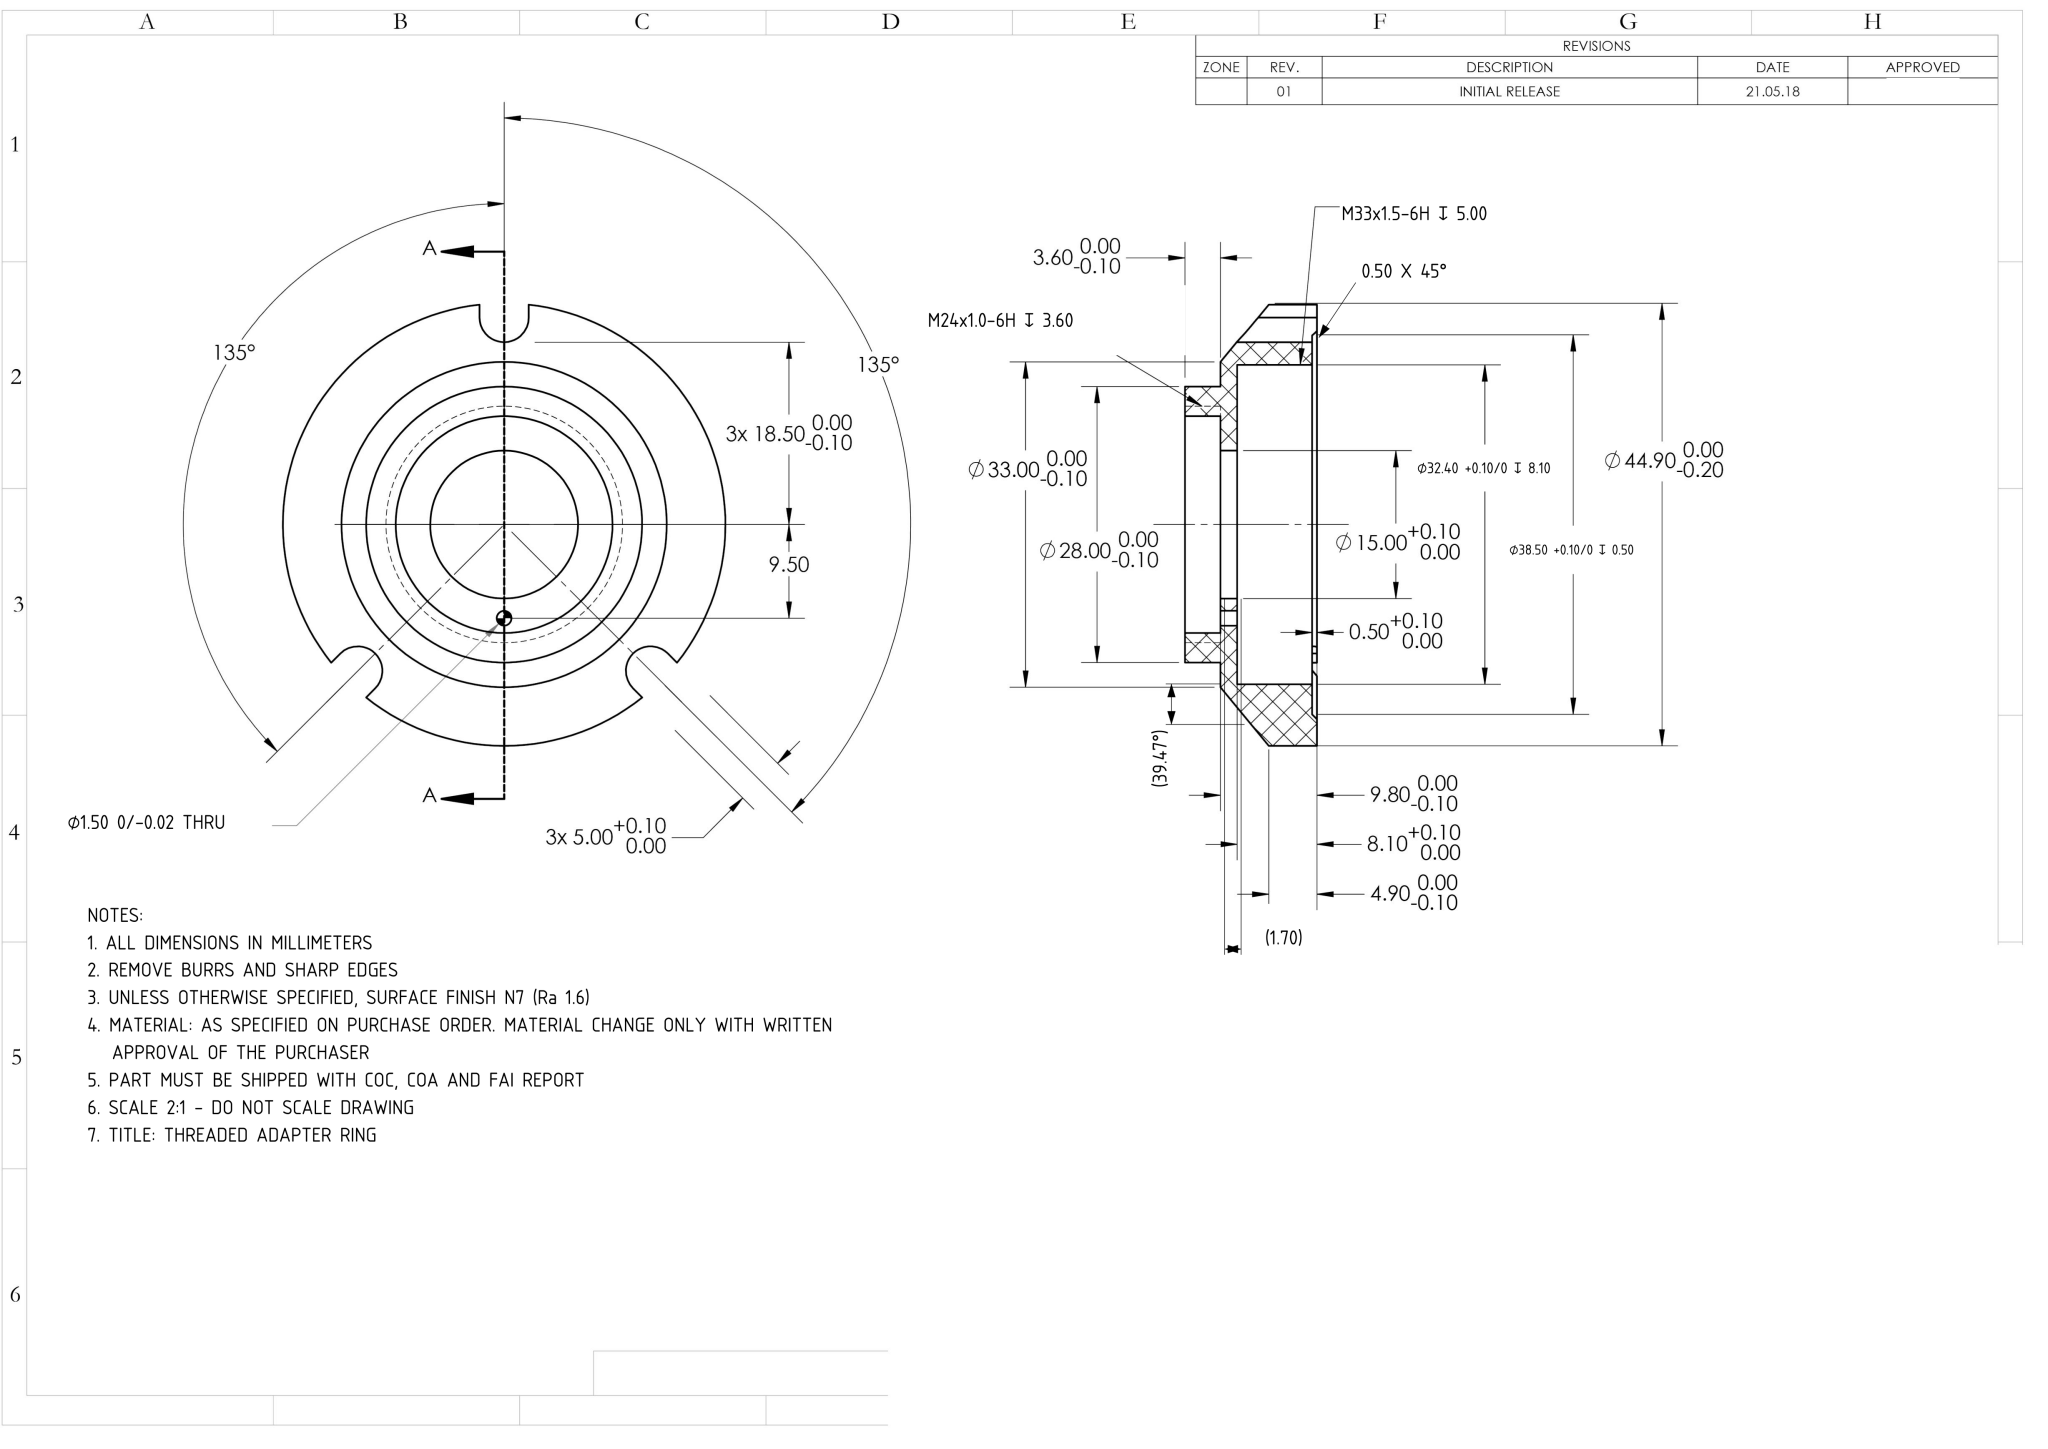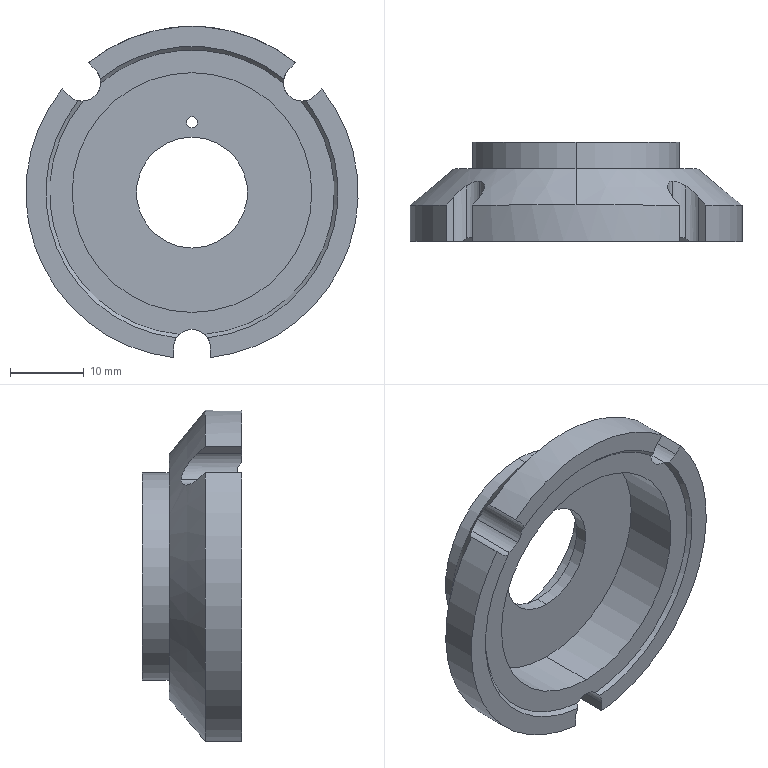Part | NX | mm | 1 solid | 40 faces | box 44.9 x 13.4 x 44.76 mm | volume 7008 mm3 | cylinder 21 | plane 14 | cone 5 | commonest cylinder face diameters 5 x8 44.9 x3 22 x2 1.5 x2 32.4 x2 15 x2 28 x2